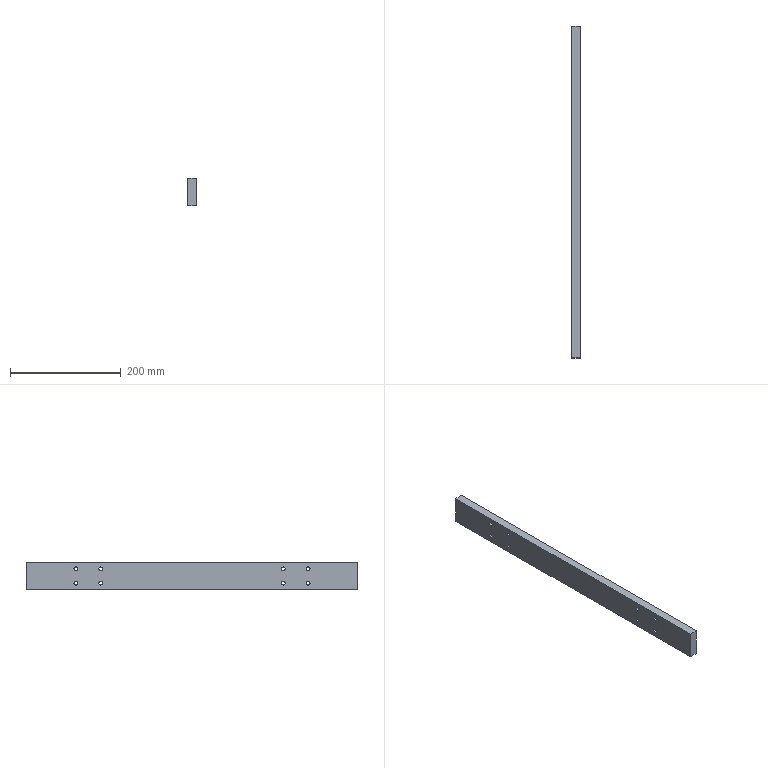Component | SolidWorks | DC-Motor-117-1 | 1 solid | 46 faces | box 15 x 600 x 50 mm | volume 442781 mm3 | cylinder 32 | plane 14 | commonest cylinder face diameters 11 x16 6.6 x16
build123d program:
from build123d import *

# Parameters (mm, degrees)
SKETCH1_W                                       = 600
SKETCH1_H                                       = 50
BOSS_EXTRUDE1_DEPTH                             = 7.5
M6_HEX_SOCKET_HEAD_CAP_SCREW_CBORE1_D           = 6.6
M6_HEX_SOCKET_HEAD_CAP_SCREW_CBORE1_CBORE_D     = 11
M6_HEX_SOCKET_HEAD_CAP_SCREW_CBORE1_CBORE_DEPTH = 6.4


with BuildPart() as part:
    # Sketch1 → Boss-Extrude1 (new, symmetric)
    with BuildSketch(Plane.XY):
        Rectangle(SKETCH1_W, SKETCH1_H)
    extrude(amount=BOSS_EXTRUDE1_DEPTH, both=True)

    # M6 Hex Socket Head Cap Screw CBORE1 (through all)
    with Locations(Plane(origin=(0, 0, -7.5), x_dir=(-1, 0, 0), z_dir=(0, 0, -1))):
        with Locations((-210, 13), (-165, 13), (-210, -13), (-165, -13), (165, 13), (210, 13), (165, -13), (210, -13)):
            CounterBoreHole(M6_HEX_SOCKET_HEAD_CAP_SCREW_CBORE1_D / 2, M6_HEX_SOCKET_HEAD_CAP_SCREW_CBORE1_CBORE_D / 2, M6_HEX_SOCKET_HEAD_CAP_SCREW_CBORE1_CBORE_DEPTH)


solid = part.part

# Placed as in the assembly
solid = solid.moved(Location((-350.292, 14.301, -463), (90, -90, 0)))